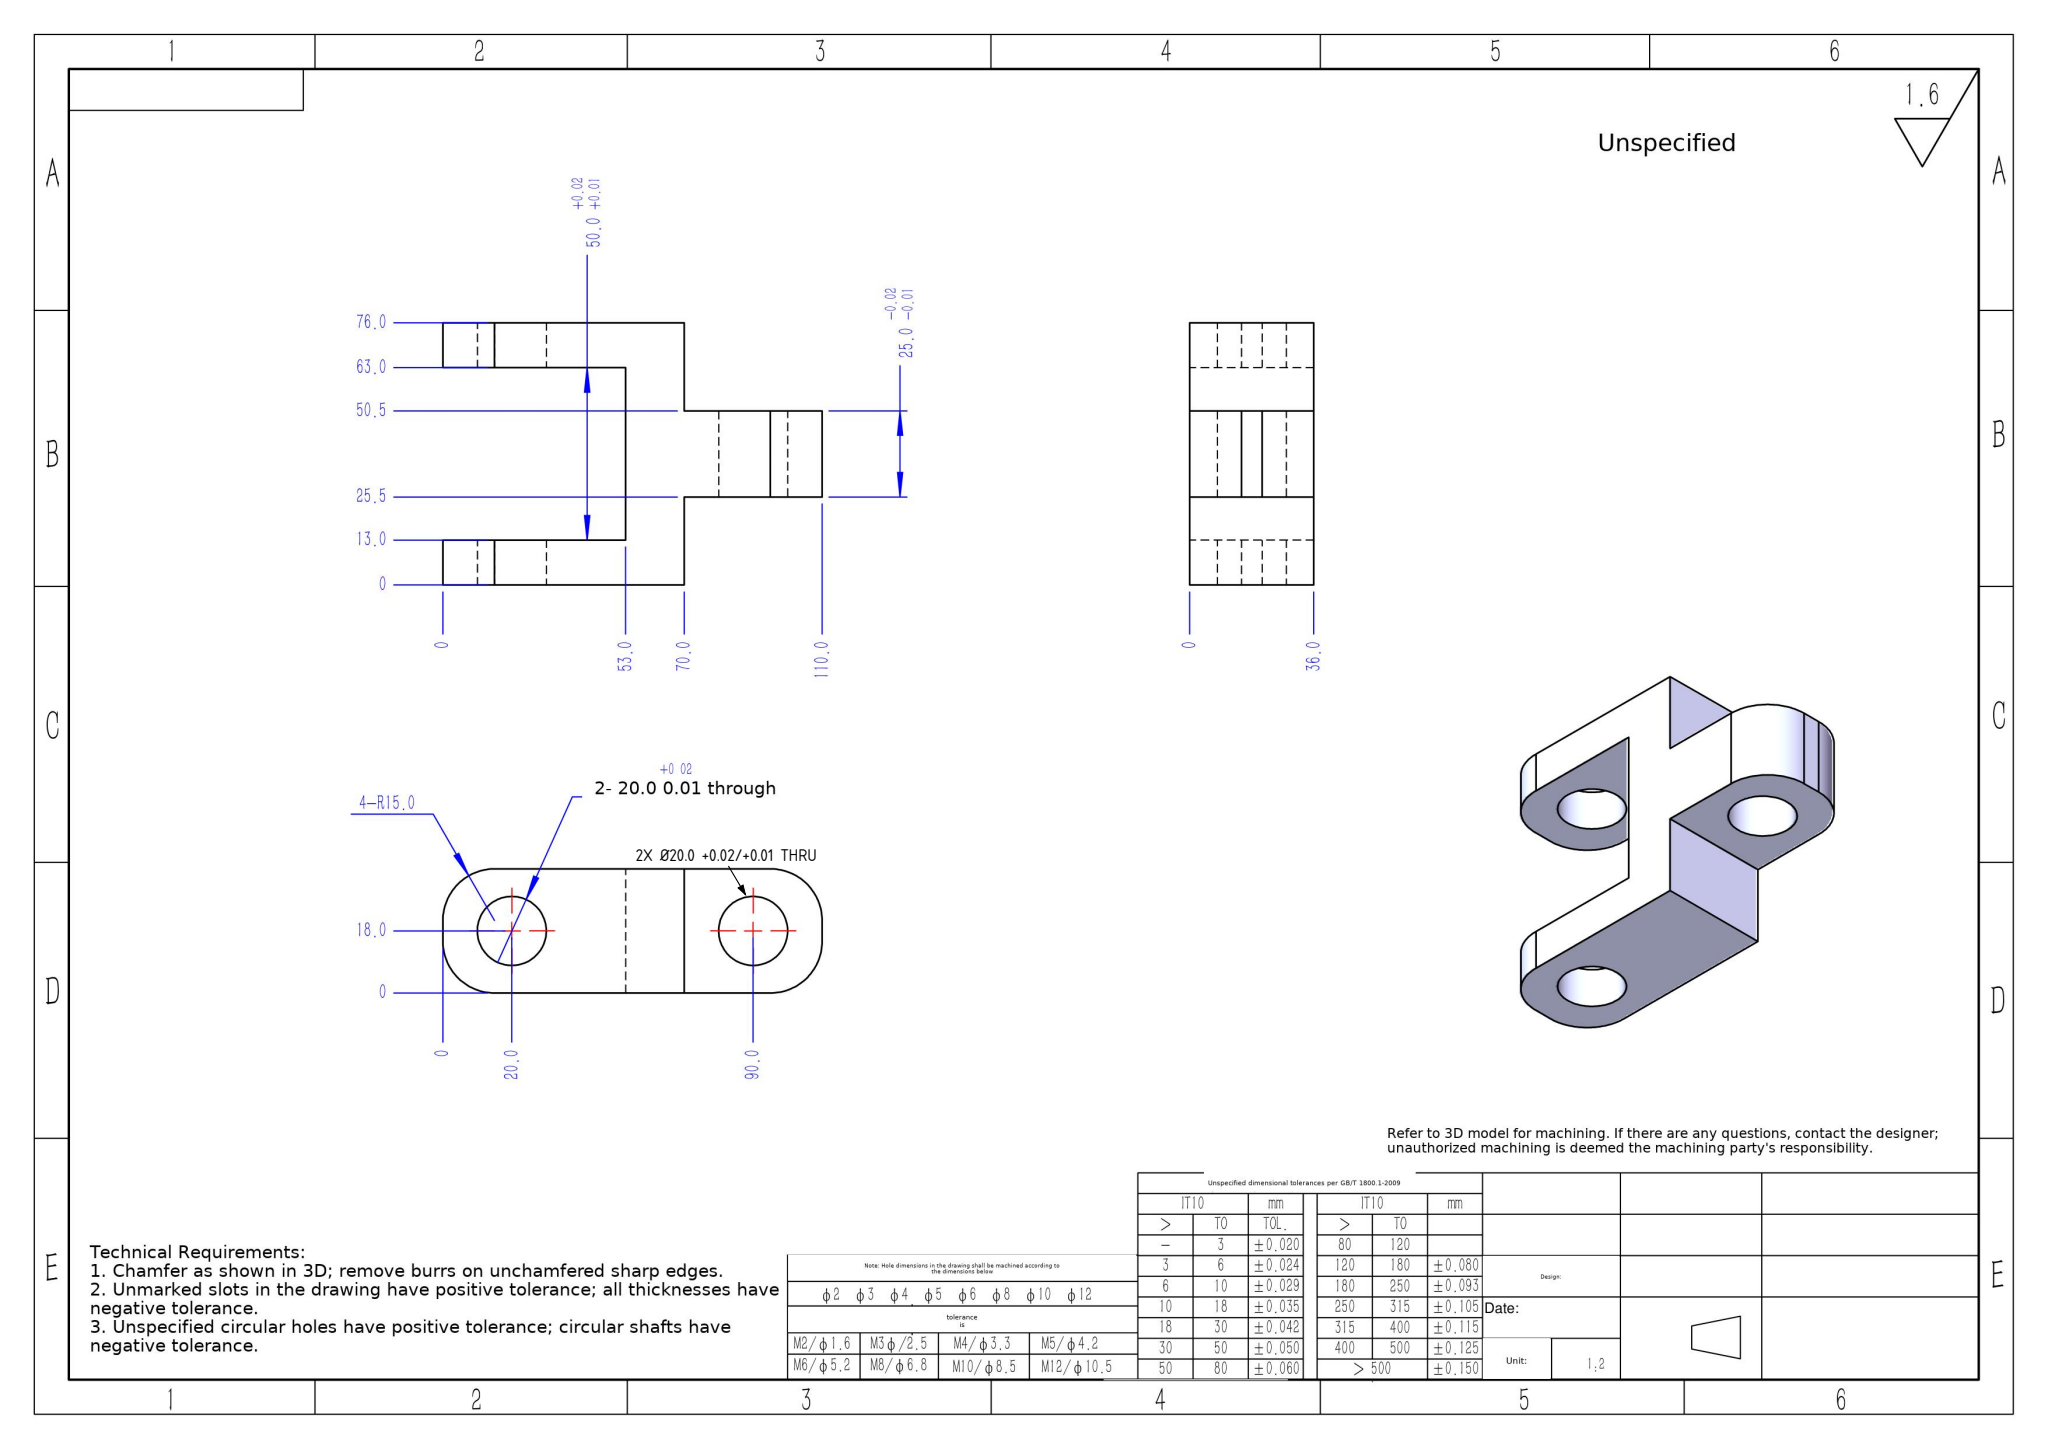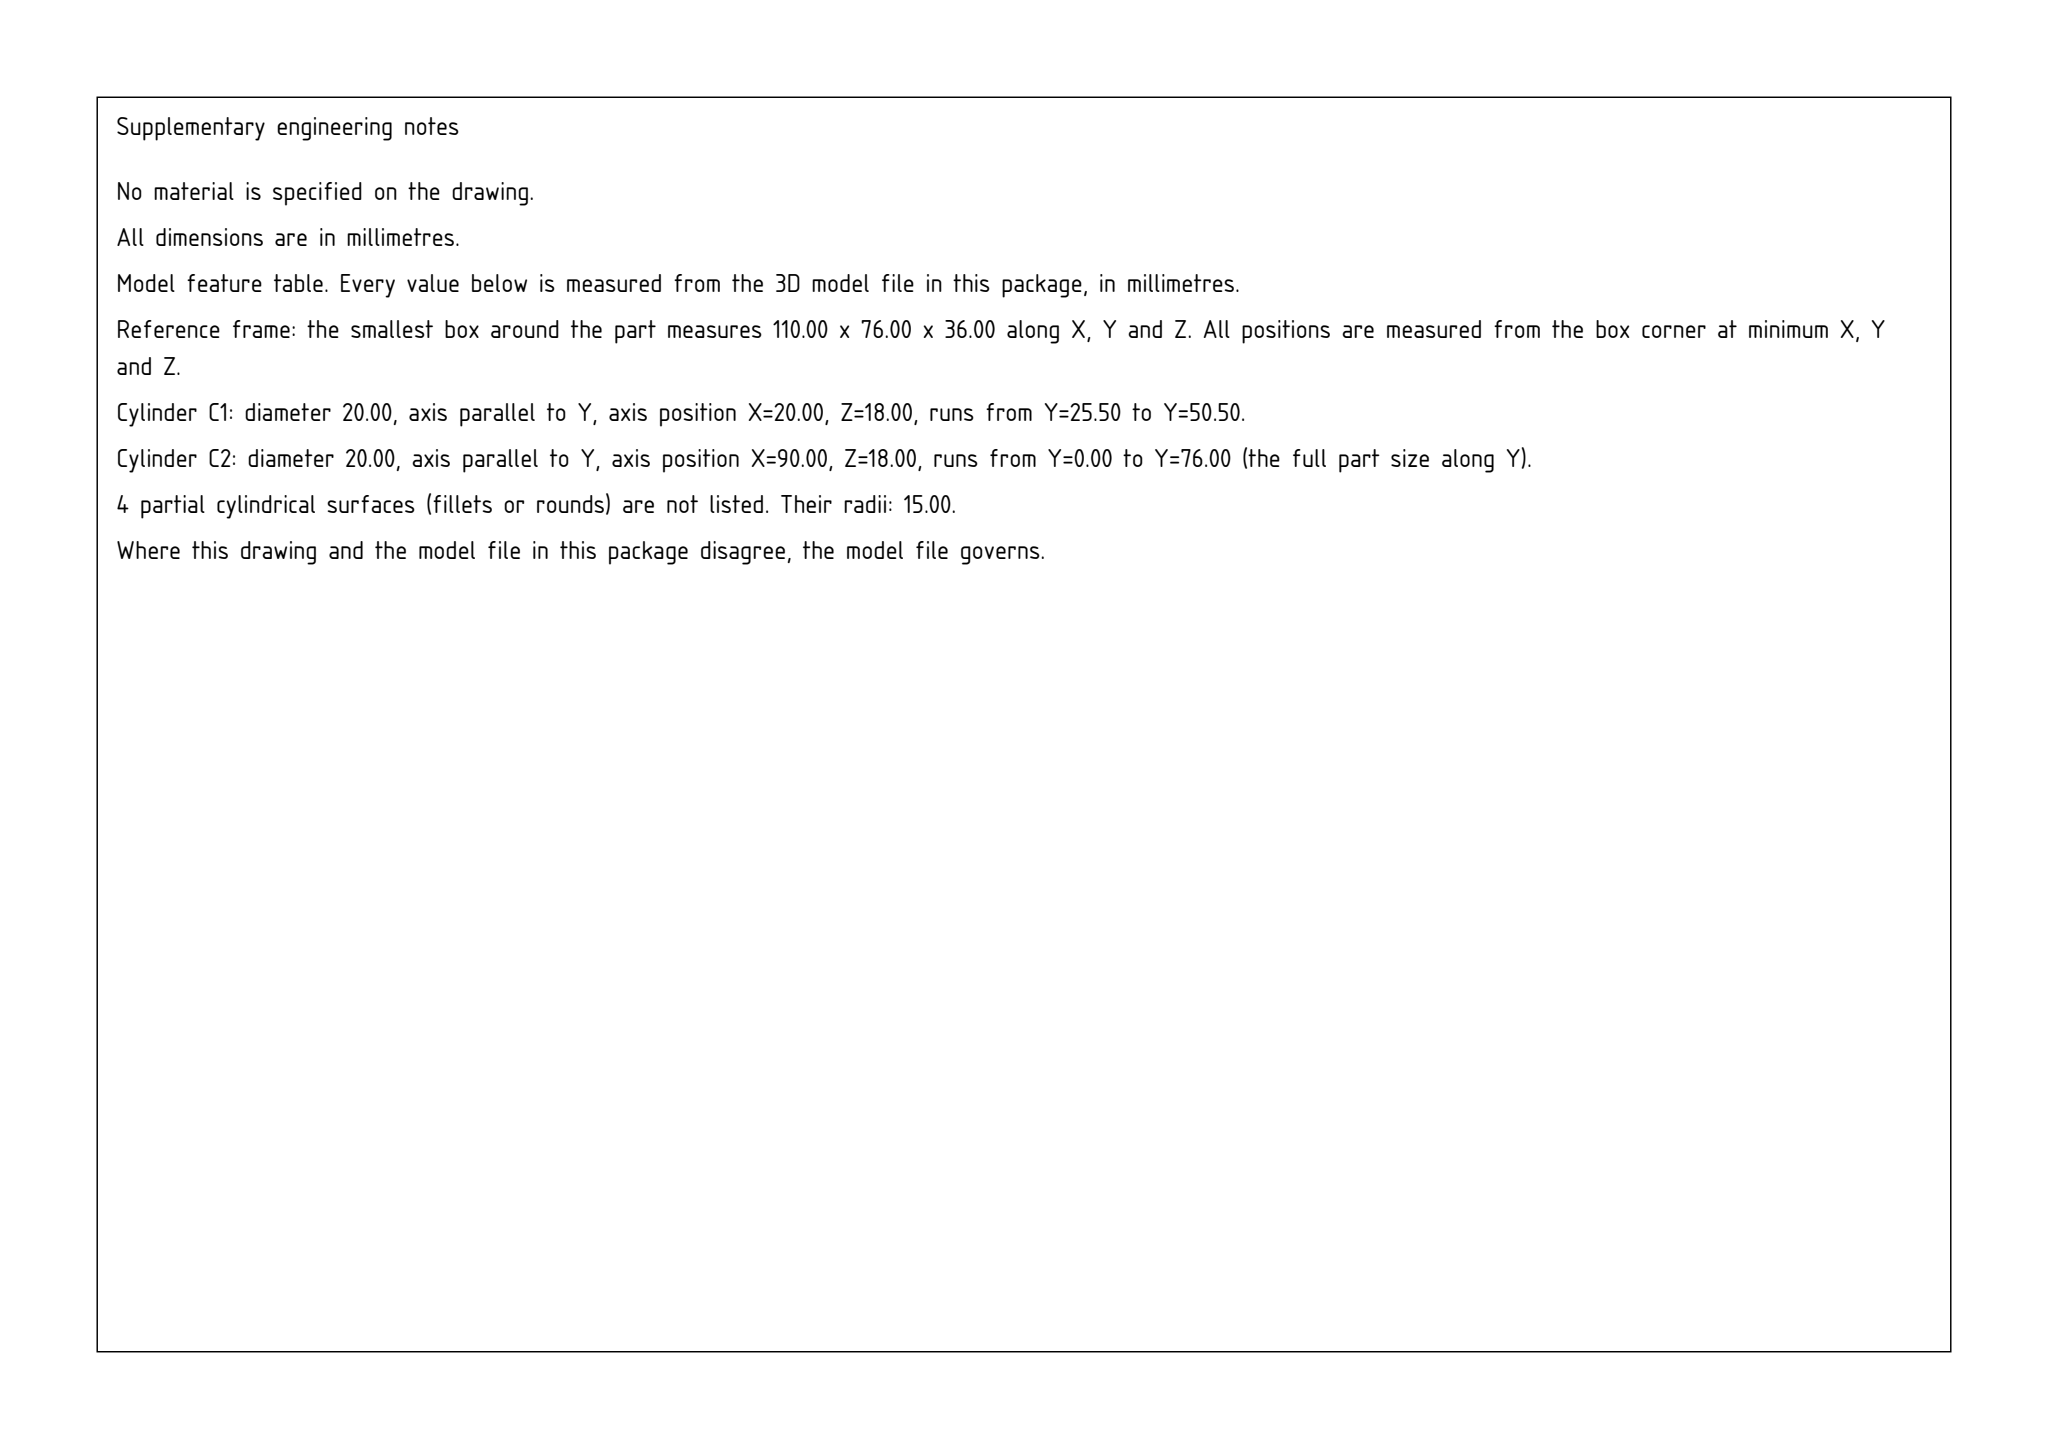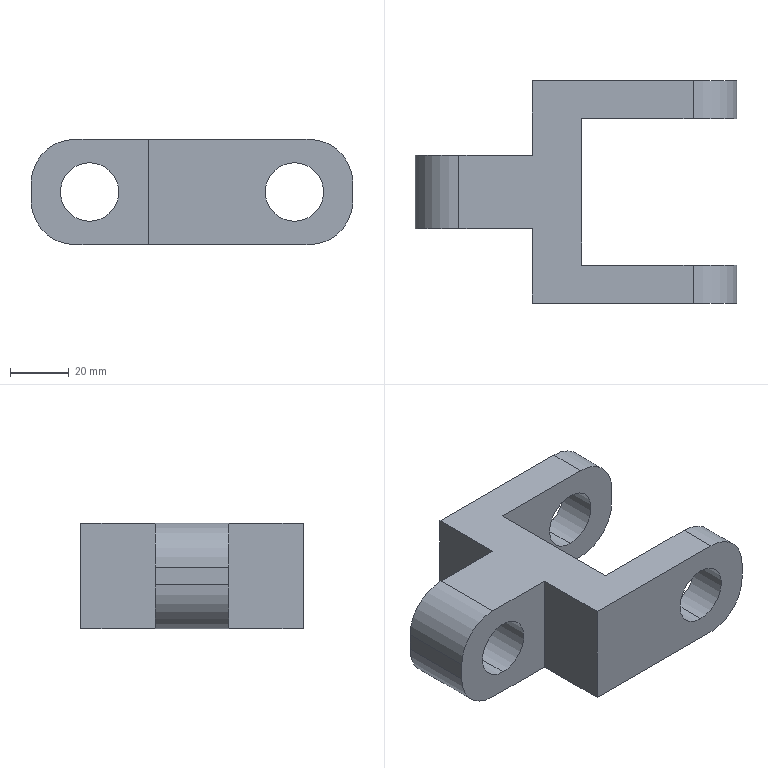Part | SolidWorks | mm | 1 solid | 26 faces | box 110 x 76 x 36 mm | volume 111173 mm3 | plane 14 | cylinder 12 | commonest cylinder face diameters 20 x6 30 x6
Drawing notes:
2X Ø20.0 +0.02/+0.01 THRU | from the solid: hole/bore dia 20.0 axis y at (x20,z18) y25.5-50.5 and (x90,z18) y0-13 & y63-76, 360 deg
build123d program:
from build123d import *

# Parameters (mm, degrees)
SKETCH1_W           = 110
SKETCH1_H           = 76
BOSS_EXTRUDE1_DEPTH = 18
SKETCH2_R           = 10
CUT_EXTRUDE1_DEPTH  = 205
SKETCH3_W           = 40
SKETCH3_H           = 36
CUT_EXTRUDE2_DEPTH  = 25.5
SKETCH4_W           = 53
SKETCH4_H           = 50
CUT_EXTRUDE3_DEPTH  = 256
FILLET1_R           = 15


with BuildPart() as part:
    # Sketch1 → Boss-Extrude1 (new, symmetric)
    with BuildSketch(Plane.XY):
        Rectangle(SKETCH1_W, SKETCH1_H)
    extrude(amount=BOSS_EXTRUDE1_DEPTH, both=True)

    # Sketch2 → Cut-Extrude1 (cut)
    with BuildSketch(Plane.XZ.offset(38)):
        with Locations(Location((35, 0, 0), (0, 0, 270))):
            Circle(SKETCH2_R)
    cut_extrude1 = extrude(amount=-CUT_EXTRUDE1_DEPTH, mode=Mode.SUBTRACT)

    # Mirror1: Cut-Extrude1 across plane
    add(cut_extrude1.mirror(Plane(origin=(0, 0, 0), x_dir=(0, 0, 1), z_dir=(1, 0, 0))), mode=Mode.SUBTRACT)

    # Sketch3 → Cut-Extrude2 (cut)
    with BuildSketch(Plane.XZ.offset(38)):
        with Locations((-35, 0)):
            Rectangle(SKETCH3_W, SKETCH3_H)
    cut_extrude2 = extrude(amount=-CUT_EXTRUDE2_DEPTH, mode=Mode.SUBTRACT)

    # Mirror2: Cut-Extrude2 across plane
    add(cut_extrude2.mirror(Plane.ZX), mode=Mode.SUBTRACT)

    # Sketch4 → Cut-Extrude3 (cut)
    with BuildSketch(Plane(origin=(0, 0, -18), x_dir=(-1, 0, 0), z_dir=(0, 0, -1))):
        with Locations((-28.5, 0)):
            Rectangle(SKETCH4_W, SKETCH4_H)
    extrude(amount=-CUT_EXTRUDE3_DEPTH, mode=Mode.SUBTRACT)

    # Fillet1
    fillet1_edges = [part.edges().sort_by_distance(p)[0] for p in [
        (55, -31.5, 18),
        (-55, 0, -18),
        (-55, 0, 18),
        (55, -31.5, -18),
        (55, 31.5, -18),
        (55, 31.5, 18),
    ]]
    fillet(fillet1_edges, radius=FILLET1_R)


solid = part.part
STEP:
#1=CARTESIAN_POINT('',(35.,-25.,-10.));
#2=VERTEX_POINT('',#1);
#3=CARTESIAN_POINT('',(35.,-25.,10.));
#4=VERTEX_POINT('',#3);
#5=CARTESIAN_POINT('',(35.,-25.,0.));
#6=DIRECTION('',(0.,1.,0.));
#7=DIRECTION('',(0.,0.,-1.));
#8=AXIS2_PLACEMENT_3D('',#5,#6,#7);
#9=CIRCLE('',#8,10.);
#10=EDGE_CURVE('',#2,#4,#9,.T.);
#11=ORIENTED_EDGE('',*,*,#10,.T.);
#12=CARTESIAN_POINT('',(35.,-38.,10.));
#13=VERTEX_POINT('',#12);
#14=CARTESIAN_POINT('',(35.,167.,10.));
#15=DIRECTION('',(0.,-1.,0.));
#16=VECTOR('',#15,1000.);
#17=LINE('',#14,#16);
#18=EDGE_CURVE('',#4,#13,#17,.T.);
#19=ORIENTED_EDGE('',*,*,#18,.T.);
#20=CARTESIAN_POINT('',(35.,-38.,-10.));
#21=VERTEX_POINT('',#20);
#22=CARTESIAN_POINT('',(35.,-38.,0.));
#23=DIRECTION('',(0.,-1.,0.));
#24=DIRECTION('',(0.,0.,-1.));
#25=AXIS2_PLACEMENT_3D('',#22,#23,#24);
#26=CIRCLE('',#25,10.);
#27=EDGE_CURVE('',#13,#21,#26,.T.);
#28=ORIENTED_EDGE('',*,*,#27,.T.);
#29=CARTESIAN_POINT('',(35.,167.,-10.));
#30=DIRECTION('',(0.,-1.,0.));
#31=VECTOR('',#30,1000.);
#32=LINE('',#29,#31);
#33=EDGE_CURVE('',#2,#21,#32,.T.);
#34=ORIENTED_EDGE('',*,*,#33,.F.);
#35=EDGE_LOOP('',(#11,#19,#28,#34));
#36=FACE_OUTER_BOUND('',#35,.T.);
#37=CARTESIAN_POINT('',(35.,167.,0.));
#38=DIRECTION('',(0.,-1.,0.));
#39=DIRECTION('',(0.,0.,-1.));
#40=AXIS2_PLACEMENT_3D('',#37,#38,#39);
#41=CYLINDRICAL_SURFACE('',#40,10.);
#42=ADVANCED_FACE('',(#36),#41,.F.);
#43=CARTESIAN_POINT('',(-35.,12.5,-10.));
#44=VERTEX_POINT('',#43);
#45=CARTESIAN_POINT('',(-35.,12.5,10.));
#46=VERTEX_POINT('',#45);
#47=CARTESIAN_POINT('',(-35.,12.5,0.));
#48=DIRECTION('',(0.,1.,0.));
#49=DIRECTION('',(0.,0.,1.));
#50=AXIS2_PLACEMENT_3D('',#47,#48,#49);
#51=CIRCLE('',#50,10.);
#52=EDGE_CURVE('',#44,#46,#51,.T.);
#53=ORIENTED_EDGE('',*,*,#52,.T.);
#54=CARTESIAN_POINT('',(-35.,-12.5,10.));
#55=VERTEX_POINT('',#54);
#56=CARTESIAN_POINT('',(-35.,167.,10.));
#57=DIRECTION('',(0.,-1.,0.));
#58=VECTOR('',#57,1000.);
#59=LINE('',#56,#58);
#60=EDGE_CURVE('',#46,#55,#59,.T.);
#61=ORIENTED_EDGE('',*,*,#60,.T.);
#62=CARTESIAN_POINT('',(-35.,-12.5,-10.));
#63=VERTEX_POINT('',#62);
#64=CARTESIAN_POINT('',(-35.,-12.5,0.));
#65=DIRECTION('',(0.,-1.,0.));
#66=DIRECTION('',(0.,0.,-1.));
#67=AXIS2_PLACEMENT_3D('',#64,#65,#66);
#68=CIRCLE('',#67,10.);
#69=EDGE_CURVE('',#55,#63,#68,.T.);
#70=ORIENTED_EDGE('',*,*,#69,.T.);
#71=CARTESIAN_POINT('',(-35.,167.,-10.));
#72=DIRECTION('',(0.,-1.,0.));
#73=VECTOR('',#72,1000.);
#74=LINE('',#71,#73);
#75=EDGE_CURVE('',#44,#63,#74,.T.);
#76=ORIENTED_EDGE('',*,*,#75,.F.);
#77=EDGE_LOOP('',(#53,#61,#70,#76));
#78=FACE_OUTER_BOUND('',#77,.T.);
#79=CARTESIAN_POINT('',(-35.,167.,0.));
#80=DIRECTION('',(0.,-1.,0.));
#81=DIRECTION('',(0.,0.,-1.));
#82=AXIS2_PLACEMENT_3D('',#79,#80,#81);
#83=CYLINDRICAL_SURFACE('',#82,10.);
#84=ADVANCED_FACE('',(#78),#83,.F.);
#85=CARTESIAN_POINT('',(35.,38.,10.));
#86=VERTEX_POINT('',#85);
#87=CARTESIAN_POINT('',(35.,38.,-10.));
#88=VERTEX_POINT('',#87);
#89=CARTESIAN_POINT('',(35.,38.,0.));
#90=DIRECTION('',(0.,-1.,0.));
#91=DIRECTION('',(0.,0.,-1.));
#92=AXIS2_PLACEMENT_3D('',#89,#90,#91);
#93=CIRCLE('',#92,10.);
#94=EDGE_CURVE('',#86,#88,#93,.T.);
#95=ORIENTED_EDGE('',*,*,#94,.F.);
#96=CARTESIAN_POINT('',(35.,25.,10.));
#97=VERTEX_POINT('',#96);
#98=CARTESIAN_POINT('',(35.,167.,10.));
#99=DIRECTION('',(0.,-1.,0.));
#100=VECTOR('',#99,1000.);
#101=LINE('',#98,#100);
#102=EDGE_CURVE('',#86,#97,#101,.T.);
#103=ORIENTED_EDGE('',*,*,#102,.T.);
#104=CARTESIAN_POINT('',(35.,25.,-10.));
#105=VERTEX_POINT('',#104);
#106=CARTESIAN_POINT('',(35.,25.,0.));
#107=DIRECTION('',(-0.,-1.,0.));
#108=DIRECTION('',(-1.,0.,0.));
#109=AXIS2_PLACEMENT_3D('',#106,#107,#108);
#110=CIRCLE('',#109,10.);
#111=EDGE_CURVE('',#97,#105,#110,.T.);
#112=ORIENTED_EDGE('',*,*,#111,.T.);
#113=CARTESIAN_POINT('',(35.,167.,-10.));
#114=DIRECTION('',(0.,-1.,0.));
#115=VECTOR('',#114,1000.);
#116=LINE('',#113,#115);
#117=EDGE_CURVE('',#88,#105,#116,.T.);
#118=ORIENTED_EDGE('',*,*,#117,.F.);
#119=EDGE_LOOP('',(#95,#103,#112,#118));
#120=FACE_OUTER_BOUND('',#119,.T.);
#121=CARTESIAN_POINT('',(35.,167.,0.));
#122=DIRECTION('',(0.,-1.,0.));
#123=DIRECTION('',(0.,0.,-1.));
#124=AXIS2_PLACEMENT_3D('',#121,#122,#123);
#125=CYLINDRICAL_SURFACE('',#124,10.);
#126=ADVANCED_FACE('',(#120),#125,.F.);
#127=CARTESIAN_POINT('',(55.,25.,3.));
#128=VERTEX_POINT('',#127);
#129=CARTESIAN_POINT('',(55.,25.,-3.));
#130=VERTEX_POINT('',#129);
#131=CARTESIAN_POINT('',(55.,25.,238.));
#132=DIRECTION('',(0.,0.,-1.));
#133=VECTOR('',#132,1000.);
#134=LINE('',#131,#133);
#135=EDGE_CURVE('',#128,#130,#134,.T.);
#136=ORIENTED_EDGE('',*,*,#135,.T.);
#137=CARTESIAN_POINT('',(55.,38.,-3.));
#138=VERTEX_POINT('',#137);
#139=CARTESIAN_POINT('',(55.,38.,-3.));
#140=DIRECTION('',(0.,1.,0.));
#141=VECTOR('',#140,1000.);
#142=LINE('',#139,#141);
#143=EDGE_CURVE('',#130,#138,#142,.T.);
#144=ORIENTED_EDGE('',*,*,#143,.T.);
#145=CARTESIAN_POINT('',(55.,38.,3.));
#146=VERTEX_POINT('',#145);
#147=CARTESIAN_POINT('',(55.,38.,18.));
#148=DIRECTION('',(0.,0.,-1.));
#149=VECTOR('',#148,1000.);
#150=LINE('',#147,#149);
#151=EDGE_CURVE('',#146,#138,#150,.T.);
#152=ORIENTED_EDGE('',*,*,#151,.F.);
#153=CARTESIAN_POINT('',(55.,-38.,3.));
#154=DIRECTION('',(0.,-1.,0.));
#155=VECTOR('',#154,1000.);
#156=LINE('',#153,#155);
#157=EDGE_CURVE('',#146,#128,#156,.T.);
#158=ORIENTED_EDGE('',*,*,#157,.T.);
#159=EDGE_LOOP('',(#136,#144,#152,#158));
#160=FACE_OUTER_BOUND('',#159,.T.);
#161=CARTESIAN_POINT('',(55.,-38.,18.));
#162=DIRECTION('',(-1.,0.,0.));
#163=DIRECTION('',(0.,0.,1.));
#164=AXIS2_PLACEMENT_3D('',#161,#162,#163);
#165=PLANE('',#164);
#166=ADVANCED_FACE('',(#160),#165,.F.);
#167=ORIENTED_EDGE('',*,*,#102,.F.);
#168=CARTESIAN_POINT('',(35.,38.,0.));
#169=DIRECTION('',(0.,-1.,0.));
#170=DIRECTION('',(0.,0.,-1.));
#171=AXIS2_PLACEMENT_3D('',#168,#169,#170);
#172=CIRCLE('',#171,10.);
#173=EDGE_CURVE('',#88,#86,#172,.T.);
#174=ORIENTED_EDGE('',*,*,#173,.F.);
#175=ORIENTED_EDGE('',*,*,#117,.T.);
#176=CARTESIAN_POINT('',(35.,25.,0.));
#177=DIRECTION('',(-0.,-1.,0.));
#178=DIRECTION('',(-1.,0.,0.));
#179=AXIS2_PLACEMENT_3D('',#176,#177,#178);
#180=CIRCLE('',#179,10.);
#181=EDGE_CURVE('',#105,#97,#180,.T.);
#182=ORIENTED_EDGE('',*,*,#181,.T.);
#183=EDGE_LOOP('',(#167,#174,#175,#182));
#184=FACE_OUTER_BOUND('',#183,.T.);
#185=CARTESIAN_POINT('',(35.,167.,0.));
#186=DIRECTION('',(0.,-1.,0.));
#187=DIRECTION('',(0.,0.,-1.));
#188=AXIS2_PLACEMENT_3D('',#185,#186,#187);
#189=CYLINDRICAL_SURFACE('',#188,10.);
#190=ADVANCED_FACE('',(#184),#189,.F.);
#191=CARTESIAN_POINT('',(-55.,12.5,3.));
#192=VERTEX_POINT('',#191);
#193=CARTESIAN_POINT('',(-55.,12.5,-3.));
#194=VERTEX_POINT('',#193);
#195=CARTESIAN_POINT('',(-55.,12.5,18.));
#196=DIRECTION('',(0.,0.,-1.));
#197=VECTOR('',#196,1000.);
#198=LINE('',#195,#197);
#199=EDGE_CURVE('',#192,#194,#198,.T.);
#200=ORIENTED_EDGE('',*,*,#199,.T.);
#201=CARTESIAN_POINT('',(-55.,-12.5,-3.));
#202=VERTEX_POINT('',#201);
#203=CARTESIAN_POINT('',(-55.,-12.5,-3.));
#204=DIRECTION('',(0.,-1.,0.));
#205=VECTOR('',#204,1000.);
#206=LINE('',#203,#205);
#207=EDGE_CURVE('',#194,#202,#206,.T.);
#208=ORIENTED_EDGE('',*,*,#207,.T.);
#209=CARTESIAN_POINT('',(-55.,-12.5,3.));
#210=VERTEX_POINT('',#209);
#211=CARTESIAN_POINT('',(-55.,-12.5,18.));
#212=DIRECTION('',(0.,0.,-1.));
#213=VECTOR('',#212,1000.);
#214=LINE('',#211,#213);
#215=EDGE_CURVE('',#210,#202,#214,.T.);
#216=ORIENTED_EDGE('',*,*,#215,.F.);
#217=CARTESIAN_POINT('',(-55.,-38.,3.));
#218=DIRECTION('',(0.,1.,0.));
#219=VECTOR('',#218,1000.);
#220=LINE('',#217,#219);
#221=EDGE_CURVE('',#210,#192,#220,.T.);
#222=ORIENTED_EDGE('',*,*,#221,.T.);
#223=EDGE_LOOP('',(#200,#208,#216,#222));
#224=FACE_OUTER_BOUND('',#223,.T.);
#225=CARTESIAN_POINT('',(-55.,-38.,18.));
#226=DIRECTION('',(1.,0.,0.));
#227=DIRECTION('',(0.,0.,-1.));
#228=AXIS2_PLACEMENT_3D('',#225,#226,#227);
#229=PLANE('',#228);
#230=ADVANCED_FACE('',(#224),#229,.F.);
#231=ORIENTED_EDGE('',*,*,#60,.F.);
#232=CARTESIAN_POINT('',(-35.,12.5,0.));
#233=DIRECTION('',(0.,1.,0.));
#234=DIRECTION('',(0.,0.,1.));
#235=AXIS2_PLACEMENT_3D('',#232,#233,#234);
#236=CIRCLE('',#235,10.);
#237=EDGE_CURVE('',#46,#44,#236,.T.);
#238=ORIENTED_EDGE('',*,*,#237,.T.);
#239=ORIENTED_EDGE('',*,*,#75,.T.);
#240=CARTESIAN_POINT('',(-35.,-12.5,0.));
#241=DIRECTION('',(0.,-1.,0.));
#242=DIRECTION('',(0.,0.,-1.));
#243=AXIS2_PLACEMENT_3D('',#240,#241,#242);
#244=CIRCLE('',#243,10.);
#245=EDGE_CURVE('',#63,#55,#244,.T.);
#246=ORIENTED_EDGE('',*,*,#245,.T.);
#247=EDGE_LOOP('',(#231,#238,#239,#246));
#248=FACE_OUTER_BOUND('',#247,.T.);
#249=CARTESIAN_POINT('',(-35.,167.,0.));
#250=DIRECTION('',(0.,-1.,0.));
#251=DIRECTION('',(0.,0.,-1.));
#252=AXIS2_PLACEMENT_3D('',#249,#250,#251);
#253=CYLINDRICAL_SURFACE('',#252,10.);
#254=ADVANCED_FACE('',(#248),#253,.F.);
#255=ORIENTED_EDGE('',*,*,#173,.T.);
#256=ORIENTED_EDGE('',*,*,#94,.T.);
#257=EDGE_LOOP('',(#255,#256));
#258=FACE_BOUND('',#257,.T.);
#259=ORIENTED_EDGE('',*,*,#151,.T.);
#260=CARTESIAN_POINT('',(40.,38.,-18.));
#261=VERTEX_POINT('',#260);
#262=CARTESIAN_POINT('',(40.,38.,-3.));
#263=DIRECTION('',(0.,1.,0.));
#264=DIRECTION('',(0.,0.,-1.));
#265=AXIS2_PLACEMENT_3D('',#262,#263,#264);
#266=CIRCLE('',#265,15.);
#267=EDGE_CURVE('',#138,#261,#266,.T.);
#268=ORIENTED_EDGE('',*,*,#267,.T.);
#269=CARTESIAN_POINT('',(-15.,38.,-18.));
#270=VERTEX_POINT('',#269);
#271=CARTESIAN_POINT('',(-55.,38.,-18.));
#272=DIRECTION('',(-1.,0.,0.));
#273=VECTOR('',#272,1000.);
#274=LINE('',#271,#273);
#275=EDGE_CURVE('',#261,#270,#274,.T.);
#276=ORIENTED_EDGE('',*,*,#275,.T.);
#277=CARTESIAN_POINT('',(-15.,38.,18.));
#278=VERTEX_POINT('',#277);
#279=CARTESIAN_POINT('',(-15.,38.,18.));
#280=DIRECTION('',(-0.,0.,1.));
#281=VECTOR('',#280,1000.);
#282=LINE('',#279,#281);
#283=EDGE_CURVE('',#270,#278,#282,.T.);
#284=ORIENTED_EDGE('',*,*,#283,.T.);
#285=CARTESIAN_POINT('',(40.,38.,18.));
#286=VERTEX_POINT('',#285);
#287=CARTESIAN_POINT('',(-55.,38.,18.));
#288=DIRECTION('',(-1.,0.,0.));
#289=VECTOR('',#288,1000.);
#290=LINE('',#287,#289);
#291=EDGE_CURVE('',#286,#278,#290,.T.);
#292=ORIENTED_EDGE('',*,*,#291,.F.);
#293=CARTESIAN_POINT('',(40.,38.,3.));
#294=DIRECTION('',(0.,1.,0.));
#295=DIRECTION('',(0.,0.,-1.));
#296=AXIS2_PLACEMENT_3D('',#293,#294,#295);
#297=CIRCLE('',#296,15.);
#298=EDGE_CURVE('',#286,#146,#297,.T.);
#299=ORIENTED_EDGE('',*,*,#298,.T.);
#300=EDGE_LOOP('',(#259,#268,#276,#284,#292,#299));
#301=FACE_OUTER_BOUND('',#300,.T.);
#302=CARTESIAN_POINT('',(-55.,38.,18.));
#303=DIRECTION('',(0.,-1.,0.));
#304=DIRECTION('',(0.,0.,-1.));
#305=AXIS2_PLACEMENT_3D('',#302,#303,#304);
#306=PLANE('',#305);
#307=ADVANCED_FACE('',(#258,#301),#306,.F.);
#308=CARTESIAN_POINT('',(-15.,12.5,18.));
#309=VERTEX_POINT('',#308);
#310=CARTESIAN_POINT('',(-40.,12.5,18.));
#311=VERTEX_POINT('',#310);
#312=CARTESIAN_POINT('',(-55.,12.5,18.));
#313=DIRECTION('',(-1.,0.,0.));
#314=VECTOR('',#313,1000.);
#315=LINE('',#312,#314);
#316=EDGE_CURVE('',#309,#311,#315,.T.);
#317=ORIENTED_EDGE('',*,*,#316,.T.);
#318=CARTESIAN_POINT('',(-40.,-12.5,18.));
#319=VERTEX_POINT('',#318);
#320=CARTESIAN_POINT('',(-40.,0.,18.));
#321=DIRECTION('',(0.,-1.,0.));
#322=VECTOR('',#321,1000.);
#323=LINE('',#320,#322);
#324=EDGE_CURVE('',#311,#319,#323,.T.);
#325=ORIENTED_EDGE('',*,*,#324,.T.);
#326=CARTESIAN_POINT('',(-15.,-12.5,18.));
#327=VERTEX_POINT('',#326);
#328=CARTESIAN_POINT('',(-55.,-12.5,18.));
#329=DIRECTION('',(-1.,0.,0.));
#330=VECTOR('',#329,1000.);
#331=LINE('',#328,#330);
#332=EDGE_CURVE('',#327,#319,#331,.T.);
#333=ORIENTED_EDGE('',*,*,#332,.F.);
#334=CARTESIAN_POINT('',(-15.,-38.,18.));
#335=VERTEX_POINT('',#334);
#336=CARTESIAN_POINT('',(-15.,-12.5,18.));
#337=DIRECTION('',(0.,-1.,0.));
#338=VECTOR('',#337,1000.);
#339=LINE('',#336,#338);
#340=EDGE_CURVE('',#327,#335,#339,.T.);
#341=ORIENTED_EDGE('',*,*,#340,.T.);
#342=CARTESIAN_POINT('',(40.,-38.,18.));
#343=VERTEX_POINT('',#342);
#344=CARTESIAN_POINT('',(-55.,-38.,18.));
#345=DIRECTION('',(1.,0.,0.));
#346=VECTOR('',#345,1000.);
#347=LINE('',#344,#346);
#348=EDGE_CURVE('',#335,#343,#347,.T.);
#349=ORIENTED_EDGE('',*,*,#348,.T.);
#350=CARTESIAN_POINT('',(40.,-25.,18.));
#351=VERTEX_POINT('',#350);
#352=CARTESIAN_POINT('',(40.,0.,18.));
#353=DIRECTION('',(0.,1.,0.));
#354=VECTOR('',#353,1000.);
#355=LINE('',#352,#354);
#356=EDGE_CURVE('',#343,#351,#355,.T.);
#357=ORIENTED_EDGE('',*,*,#356,.T.);
#358=CARTESIAN_POINT('',(2.,-25.,18.));
#359=VERTEX_POINT('',#358);
#360=CARTESIAN_POINT('',(0.,-25.,18.));
#361=DIRECTION('',(-1.,0.,0.));
#362=VECTOR('',#361,1000.);
#363=LINE('',#360,#362);
#364=EDGE_CURVE('',#351,#359,#363,.T.);
#365=ORIENTED_EDGE('',*,*,#364,.T.);
#366=CARTESIAN_POINT('',(2.,25.,18.));
#367=VERTEX_POINT('',#366);
#368=CARTESIAN_POINT('',(2.,-0.,18.));
#369=DIRECTION('',(0.,1.,0.));
#370=VECTOR('',#369,1000.);
#371=LINE('',#368,#370);
#372=EDGE_CURVE('',#359,#367,#371,.T.);
#373=ORIENTED_EDGE('',*,*,#372,.T.);
#374=CARTESIAN_POINT('',(40.,25.,18.));
#375=VERTEX_POINT('',#374);
#376=CARTESIAN_POINT('',(0.,25.,18.));
#377=DIRECTION('',(1.,-0.,0.));
#378=VECTOR('',#377,1000.);
#379=LINE('',#376,#378);
#380=EDGE_CURVE('',#367,#375,#379,.T.);
#381=ORIENTED_EDGE('',*,*,#380,.T.);
#382=CARTESIAN_POINT('',(40.,0.,18.));
#383=DIRECTION('',(0.,1.,0.));
#384=VECTOR('',#383,1000.);
#385=LINE('',#382,#384);
#386=EDGE_CURVE('',#375,#286,#385,.T.);
#387=ORIENTED_EDGE('',*,*,#386,.T.);
#388=ORIENTED_EDGE('',*,*,#291,.T.);
#389=CARTESIAN_POINT('',(-15.,12.5,18.));
#390=DIRECTION('',(0.,1.,0.));
#391=VECTOR('',#390,1000.);
#392=LINE('',#389,#391);
#393=EDGE_CURVE('',#309,#278,#392,.T.);
#394=ORIENTED_EDGE('',*,*,#393,.F.);
#395=EDGE_LOOP('',(#317,#325,#333,#341,#349,#357,#365,#373,#381,#387,#388,#394));
#396=FACE_OUTER_BOUND('',#395,.T.);
#397=CARTESIAN_POINT('',(0.,0.,18.));
#398=DIRECTION('',(0.,0.,-1.));
#399=DIRECTION('',(-1.,0.,0.));
#400=AXIS2_PLACEMENT_3D('',#397,#398,#399);
#401=PLANE('',#400);
#402=ADVANCED_FACE('',(#396),#401,.F.);
#403=CARTESIAN_POINT('',(-40.,-12.5,-18.));
#404=VERTEX_POINT('',#403);
#405=CARTESIAN_POINT('',(-15.,-12.5,-18.));
#406=VERTEX_POINT('',#405);
#407=CARTESIAN_POINT('',(-55.,-12.5,-18.));
#408=DIRECTION('',(1.,0.,0.));
#409=VECTOR('',#408,1000.);
#410=LINE('',#407,#409);
#411=EDGE_CURVE('',#404,#406,#410,.T.);
#412=ORIENTED_EDGE('',*,*,#411,.F.);
#413=CARTESIAN_POINT('',(-40.,12.5,-18.));
#414=VERTEX_POINT('',#413);
#415=CARTESIAN_POINT('',(-40.,12.5,-18.));
#416=DIRECTION('',(0.,1.,0.));
#417=VECTOR('',#416,1000.);
#418=LINE('',#415,#417);
#419=EDGE_CURVE('',#404,#414,#418,.T.);
#420=ORIENTED_EDGE('',*,*,#419,.T.);
#421=CARTESIAN_POINT('',(-15.,12.5,-18.));
#422=VERTEX_POINT('',#421);
#423=CARTESIAN_POINT('',(-55.,12.5,-18.));
#424=DIRECTION('',(1.,0.,0.));
#425=VECTOR('',#424,1000.);
#426=LINE('',#423,#425);
#427=EDGE_CURVE('',#414,#422,#426,.T.);
#428=ORIENTED_EDGE('',*,*,#427,.T.);
#429=CARTESIAN_POINT('',(-15.,12.5,-18.));
#430=DIRECTION('',(0.,1.,0.));
#431=VECTOR('',#430,1000.);
#432=LINE('',#429,#431);
#433=EDGE_CURVE('',#422,#270,#432,.T.);
#434=ORIENTED_EDGE('',*,*,#433,.T.);
#435=ORIENTED_EDGE('',*,*,#275,.F.);
#436=CARTESIAN_POINT('',(40.,25.,-18.));
#437=VERTEX_POINT('',#436);
#438=CARTESIAN_POINT('',(40.,25.,-18.));
#439=DIRECTION('',(0.,-1.,0.));
#440=VECTOR('',#439,1000.);
#441=LINE('',#438,#440);
#442=EDGE_CURVE('',#261,#437,#441,.T.);
#443=ORIENTED_EDGE('',*,*,#442,.T.);
#444=CARTESIAN_POINT('',(2.,25.,-18.));
#445=VERTEX_POINT('',#444);
#446=CARTESIAN_POINT('',(55.,25.,-18.));
#447=DIRECTION('',(1.,-0.,0.));
#448=VECTOR('',#447,1000.);
#449=LINE('',#446,#448);
#450=EDGE_CURVE('',#445,#437,#449,.T.);
#451=ORIENTED_EDGE('',*,*,#450,.F.);
#452=CARTESIAN_POINT('',(2.,-25.,-18.));
#453=VERTEX_POINT('',#452);
#454=CARTESIAN_POINT('',(2.,-25.,-18.));
#455=DIRECTION('',(0.,1.,0.));
#456=VECTOR('',#455,1000.);
#457=LINE('',#454,#456);
#458=EDGE_CURVE('',#453,#445,#457,.T.);
#459=ORIENTED_EDGE('',*,*,#458,.F.);
#460=CARTESIAN_POINT('',(40.,-25.,-18.));
#461=VERTEX_POINT('',#460);
#462=CARTESIAN_POINT('',(55.,-25.,-18.));
#463=DIRECTION('',(-1.,0.,0.));
#464=VECTOR('',#463,1000.);
#465=LINE('',#462,#464);
#466=EDGE_CURVE('',#461,#453,#465,.T.);
#467=ORIENTED_EDGE('',*,*,#466,.F.);
#468=CARTESIAN_POINT('',(40.,-38.,-18.));
#469=VERTEX_POINT('',#468);
#470=CARTESIAN_POINT('',(40.,-38.,-18.));
#471=DIRECTION('',(0.,-1.,0.));
#472=VECTOR('',#471,1000.);
#473=LINE('',#470,#472);
#474=EDGE_CURVE('',#461,#469,#473,.T.);
#475=ORIENTED_EDGE('',*,*,#474,.T.);
#476=CARTESIAN_POINT('',(-15.,-38.,-18.));
#477=VERTEX_POINT('',#476);
#478=CARTESIAN_POINT('',(-55.,-38.,-18.));
#479=DIRECTION('',(1.,0.,0.));
#480=VECTOR('',#479,1000.);
#481=LINE('',#478,#480);
#482=EDGE_CURVE('',#477,#469,#481,.T.);
#483=ORIENTED_EDGE('',*,*,#482,.F.);
#484=CARTESIAN_POINT('',(-15.,-12.5,-18.));
#485=DIRECTION('',(0.,-1.,0.));
#486=VECTOR('',#485,1000.);
#487=LINE('',#484,#486);
#488=EDGE_CURVE('',#406,#477,#487,.T.);
#489=ORIENTED_EDGE('',*,*,#488,.F.);
#490=EDGE_LOOP('',(#412,#420,#428,#434,#435,#443,#451,#459,#467,#475,#483,#489));
#491=FACE_OUTER_BOUND('',#490,.T.);
#492=CARTESIAN_POINT('',(0.,0.,-18.));
#493=DIRECTION('',(0.,0.,-1.));
#494=DIRECTION('',(-1.,0.,0.));
#495=AXIS2_PLACEMENT_3D('',#492,#493,#494);
#496=PLANE('',#495);
#497=ADVANCED_FACE('',(#491),#496,.T.);
#498=CARTESIAN_POINT('',(55.,-38.,3.));
#499=VERTEX_POINT('',#498);
#500=CARTESIAN_POINT('',(55.,-38.,-3.));
#501=VERTEX_POINT('',#500);
#502=CARTESIAN_POINT('',(55.,-38.,18.));
#503=DIRECTION('',(0.,0.,-1.));
#504=VECTOR('',#503,1000.);
#505=LINE('',#502,#504);
#506=EDGE_CURVE('',#499,#501,#505,.T.);
#507=ORIENTED_EDGE('',*,*,#506,.T.);
#508=CARTESIAN_POINT('',(55.,-25.,-3.));
#509=VERTEX_POINT('',#508);
#510=CARTESIAN_POINT('',(55.,-25.,-3.));
#511=DIRECTION('',(0.,1.,0.));
#512=VECTOR('',#511,1000.);
#513=LINE('',#510,#512);
#514=EDGE_CURVE('',#501,#509,#513,.T.);
#515=ORIENTED_EDGE('',*,*,#514,.T.);
#516=CARTESIAN_POINT('',(55.,-25.,3.));
#517=VERTEX_POINT('',#516);
#518=CARTESIAN_POINT('',(55.,-25.,238.));
#519=DIRECTION('',(0.,0.,-1.));
#520=VECTOR('',#519,1000.);
#521=LINE('',#518,#520);
#522=EDGE_CURVE('',#517,#509,#521,.T.);
#523=ORIENTED_EDGE('',*,*,#522,.F.);
#524=CARTESIAN_POINT('',(55.,-38.,3.));
#525=DIRECTION('',(0.,-1.,0.));
#526=VECTOR('',#525,1000.);
#527=LINE('',#524,#526);
#528=EDGE_CURVE('',#517,#499,#527,.T.);
#529=ORIENTED_EDGE('',*,*,#528,.T.);
#530=EDGE_LOOP('',(#507,#515,#523,#529));
#531=FACE_OUTER_BOUND('',#530,.T.);
#532=CARTESIAN_POINT('',(55.,-38.,18.));
#533=DIRECTION('',(-1.,0.,0.));
#534=DIRECTION('',(0.,0.,1.));
#535=AXIS2_PLACEMENT_3D('',#532,#533,#534);
#536=PLANE('',#535);
#537=ADVANCED_FACE('',(#531),#536,.F.);
#538=CARTESIAN_POINT('',(35.,-38.,0.));
#539=DIRECTION('',(0.,-1.,0.));
#540=DIRECTION('',(0.,0.,-1.));
#541=AXIS2_PLACEMENT_3D('',#538,#539,#540);
#542=CIRCLE('',#541,10.);
#543=EDGE_CURVE('',#21,#13,#542,.T.);
#544=ORIENTED_EDGE('',*,*,#543,.F.);
#545=ORIENTED_EDGE('',*,*,#27,.F.);
#546=EDGE_LOOP('',(#544,#545));
#547=FACE_BOUND('',#546,.T.);
#548=ORIENTED_EDGE('',*,*,#482,.T.);
#549=CARTESIAN_POINT('',(40.,-38.,-3.));
#550=DIRECTION('',(0.,-1.,0.));
#551=DIRECTION('',(0.,0.,1.));
#552=AXIS2_PLACEMENT_3D('',#549,#550,#551);
#553=CIRCLE('',#552,15.);
#554=EDGE_CURVE('',#469,#501,#553,.T.);
#555=ORIENTED_EDGE('',*,*,#554,.T.);
#556=ORIENTED_EDGE('',*,*,#506,.F.);
#557=CARTESIAN_POINT('',(40.,-38.,3.));
#558=DIRECTION('',(0.,-1.,0.));
#559=DIRECTION('',(0.,0.,1.));
#560=AXIS2_PLACEMENT_3D('',#557,#558,#559);
#561=CIRCLE('',#560,15.);
#562=EDGE_CURVE('',#499,#343,#561,.T.);
#563=ORIENTED_EDGE('',*,*,#562,.T.);
#564=ORIENTED_EDGE('',*,*,#348,.F.);
#565=CARTESIAN_POINT('',(-15.,-38.,18.));
#566=DIRECTION('',(-0.,0.,1.));
#567=VECTOR('',#566,1000.);
#568=LINE('',#565,#567);
#569=EDGE_CURVE('',#477,#335,#568,.T.);
#570=ORIENTED_EDGE('',*,*,#569,.F.);
#571=EDGE_LOOP('',(#548,#555,#556,#563,#564,#570));
#572=FACE_OUTER_BOUND('',#571,.T.);
#573=CARTESIAN_POINT('',(-55.,-38.,18.));
#574=DIRECTION('',(0.,1.,0.));
#575=DIRECTION('',(0.,0.,1.));
#576=AXIS2_PLACEMENT_3D('',#573,#574,#575);
#577=PLANE('',#576);
#578=ADVANCED_FACE('',(#547,#572),#577,.F.);
#579=ORIENTED_EDGE('',*,*,#18,.F.);
#580=CARTESIAN_POINT('',(35.,-25.,0.));
#581=DIRECTION('',(0.,1.,0.));
#582=DIRECTION('',(0.,0.,-1.));
#583=AXIS2_PLACEMENT_3D('',#580,#581,#582);
#584=CIRCLE('',#583,10.);
#585=EDGE_CURVE('',#4,#2,#584,.T.);
#586=ORIENTED_EDGE('',*,*,#585,.T.);
#587=ORIENTED_EDGE('',*,*,#33,.T.);
#588=ORIENTED_EDGE('',*,*,#543,.T.);
#589=EDGE_LOOP('',(#579,#586,#587,#588));
#590=FACE_OUTER_BOUND('',#589,.T.);
#591=CARTESIAN_POINT('',(35.,167.,0.));
#592=DIRECTION('',(0.,-1.,0.));
#593=DIRECTION('',(0.,0.,-1.));
#594=AXIS2_PLACEMENT_3D('',#591,#592,#593);
#595=CYLINDRICAL_SURFACE('',#594,10.);
#596=ADVANCED_FACE('',(#590),#595,.F.);
#597=ORIENTED_EDGE('',*,*,#569,.T.);
#598=ORIENTED_EDGE('',*,*,#340,.F.);
#599=CARTESIAN_POINT('',(-15.,-12.5,18.));
#600=DIRECTION('',(-0.,0.,1.));
#601=VECTOR('',#600,1000.);
#602=LINE('',#599,#601);
#603=EDGE_CURVE('',#406,#327,#602,.T.);
#604=ORIENTED_EDGE('',*,*,#603,.F.);
#605=ORIENTED_EDGE('',*,*,#488,.T.);
#606=EDGE_LOOP('',(#597,#598,#604,#605));
#607=FACE_OUTER_BOUND('',#606,.T.);
#608=CARTESIAN_POINT('',(-15.,-12.5,18.));
#609=DIRECTION('',(1.,0.,0.));
#610=DIRECTION('',(0.,0.,-1.));
#611=AXIS2_PLACEMENT_3D('',#608,#609,#610);
#612=PLANE('',#611);
#613=ADVANCED_FACE('',(#607),#612,.F.);
#614=ORIENTED_EDGE('',*,*,#245,.F.);
#615=ORIENTED_EDGE('',*,*,#69,.F.);
#616=EDGE_LOOP('',(#614,#615));
#617=FACE_BOUND('',#616,.T.);
#618=ORIENTED_EDGE('',*,*,#215,.T.);
#619=CARTESIAN_POINT('',(-40.,-12.5,-3.));
#620=DIRECTION('',(0.,-1.,0.));
#621=DIRECTION('',(0.,0.,-1.));
#622=AXIS2_PLACEMENT_3D('',#619,#620,#621);
#623=CIRCLE('',#622,15.);
#624=EDGE_CURVE('',#202,#404,#623,.T.);
#625=ORIENTED_EDGE('',*,*,#624,.T.);
#626=ORIENTED_EDGE('',*,*,#411,.T.);
#627=ORIENTED_EDGE('',*,*,#603,.T.);
#628=ORIENTED_EDGE('',*,*,#332,.T.);
#629=CARTESIAN_POINT('',(-40.,-12.5,3.));
#630=DIRECTION('',(0.,-1.,0.));
#631=DIRECTION('',(0.,0.,-1.));
#632=AXIS2_PLACEMENT_3D('',#629,#630,#631);
#633=CIRCLE('',#632,15.);
#634=EDGE_CURVE('',#319,#210,#633,.T.);
#635=ORIENTED_EDGE('',*,*,#634,.T.);
#636=EDGE_LOOP('',(#618,#625,#626,#627,#628,#635));
#637=FACE_OUTER_BOUND('',#636,.T.);
#638=CARTESIAN_POINT('',(0.,-12.5,0.));
#639=DIRECTION('',(0.,-1.,0.));
#640=DIRECTION('',(0.,0.,-1.));
#641=AXIS2_PLACEMENT_3D('',#638,#639,#640);
#642=PLANE('',#641);
#643=ADVANCED_FACE('',(#617,#637),#642,.T.);
#644=ORIENTED_EDGE('',*,*,#283,.F.);
#645=ORIENTED_EDGE('',*,*,#433,.F.);
#646=CARTESIAN_POINT('',(-15.,12.5,18.));
#647=DIRECTION('',(-0.,0.,1.));
#648=VECTOR('',#647,1000.);
#649=LINE('',#646,#648);
#650=EDGE_CURVE('',#422,#309,#649,.T.);
#651=ORIENTED_EDGE('',*,*,#650,.T.);
#652=ORIENTED_EDGE('',*,*,#393,.T.);
#653=EDGE_LOOP('',(#644,#645,#651,#652));
#654=FACE_OUTER_BOUND('',#653,.T.);
#655=CARTESIAN_POINT('',(-15.,12.5,18.));
#656=DIRECTION('',(-1.,0.,-0.));
#657=DIRECTION('',(-0.,0.,1.));
#658=AXIS2_PLACEMENT_3D('',#655,#656,#657);
#659=PLANE('',#658);
#660=ADVANCED_FACE('',(#654),#659,.T.);
#661=ORIENTED_EDGE('',*,*,#52,.F.);
#662=ORIENTED_EDGE('',*,*,#237,.F.);
#663=EDGE_LOOP('',(#661,#662));
#664=FACE_BOUND('',#663,.T.);
#665=ORIENTED_EDGE('',*,*,#427,.F.);
#666=CARTESIAN_POINT('',(-40.,12.5,-3.));
#667=DIRECTION('',(0.,1.,0.));
#668=DIRECTION('',(0.,0.,1.));
#669=AXIS2_PLACEMENT_3D('',#666,#667,#668);
#670=CIRCLE('',#669,15.);
#671=EDGE_CURVE('',#414,#194,#670,.T.);
#672=ORIENTED_EDGE('',*,*,#671,.T.);
#673=ORIENTED_EDGE('',*,*,#199,.F.);
#674=CARTESIAN_POINT('',(-40.,12.5,3.));
#675=DIRECTION('',(0.,1.,0.));
#676=DIRECTION('',(0.,0.,1.));
#677=AXIS2_PLACEMENT_3D('',#674,#675,#676);
#678=CIRCLE('',#677,15.);
#679=EDGE_CURVE('',#192,#311,#678,.T.);
#680=ORIENTED_EDGE('',*,*,#679,.T.);
#681=ORIENTED_EDGE('',*,*,#316,.F.);
#682=ORIENTED_EDGE('',*,*,#650,.F.);
#683=EDGE_LOOP('',(#665,#672,#673,#680,#681,#682));
#684=FACE_OUTER_BOUND('',#683,.T.);
#685=CARTESIAN_POINT('',(0.,12.5,0.));
#686=DIRECTION('',(0.,1.,0.));
#687=DIRECTION('',(0.,0.,-1.));
#688=AXIS2_PLACEMENT_3D('',#685,#686,#687);
#689=PLANE('',#688);
#690=ADVANCED_FACE('',(#664,#684),#689,.T.);
#691=CARTESIAN_POINT('',(2.,-25.,238.));
#692=DIRECTION('',(0.,0.,-1.));
#693=VECTOR('',#692,1000.);
#694=LINE('',#691,#693);
#695=EDGE_CURVE('',#359,#453,#694,.T.);
#696=ORIENTED_EDGE('',*,*,#695,.T.);
#697=ORIENTED_EDGE('',*,*,#458,.T.);
#698=CARTESIAN_POINT('',(2.,25.,238.));
#699=DIRECTION('',(0.,0.,-1.));
#700=VECTOR('',#699,1000.);
#701=LINE('',#698,#700);
#702=EDGE_CURVE('',#367,#445,#701,.T.);
#703=ORIENTED_EDGE('',*,*,#702,.F.);
#704=ORIENTED_EDGE('',*,*,#372,.F.);
#705=EDGE_LOOP('',(#696,#697,#703,#704));
#706=FACE_OUTER_BOUND('',#705,.T.);
#707=CARTESIAN_POINT('',(2.,-25.,238.));
#708=DIRECTION('',(-1.,0.,0.));
#709=DIRECTION('',(-0.,-1.,0.));
#710=AXIS2_PLACEMENT_3D('',#707,#708,#709);
#711=PLANE('',#710);
#712=ADVANCED_FACE('',(#706),#711,.F.);
#713=ORIENTED_EDGE('',*,*,#181,.F.);
#714=ORIENTED_EDGE('',*,*,#111,.F.);
#715=EDGE_LOOP('',(#713,#714));
#716=FACE_BOUND('',#715,.T.);
#717=ORIENTED_EDGE('',*,*,#450,.T.);
#718=CARTESIAN_POINT('',(40.,25.,-3.));
#719=DIRECTION('',(-0.,-1.,0.));
#720=DIRECTION('',(-1.,0.,0.));
#721=AXIS2_PLACEMENT_3D('',#718,#719,#720);
#722=CIRCLE('',#721,15.);
#723=EDGE_CURVE('',#437,#130,#722,.T.);
#724=ORIENTED_EDGE('',*,*,#723,.T.);
#725=ORIENTED_EDGE('',*,*,#135,.F.);
#726=CARTESIAN_POINT('',(40.,25.,3.));
#727=DIRECTION('',(-0.,-1.,0.));
#728=DIRECTION('',(-1.,0.,0.));
#729=AXIS2_PLACEMENT_3D('',#726,#727,#728);
#730=CIRCLE('',#729,15.);
#731=EDGE_CURVE('',#128,#375,#730,.T.);
#732=ORIENTED_EDGE('',*,*,#731,.T.);
#733=ORIENTED_EDGE('',*,*,#380,.F.);
#734=ORIENTED_EDGE('',*,*,#702,.T.);
#735=EDGE_LOOP('',(#717,#724,#725,#732,#733,#734));
#736=FACE_OUTER_BOUND('',#735,.T.);
#737=CARTESIAN_POINT('',(55.,25.,238.));
#738=DIRECTION('',(0.,1.,0.));
#739=DIRECTION('',(-1.,0.,0.));
#740=AXIS2_PLACEMENT_3D('',#737,#738,#739);
#741=PLANE('',#740);
#742=ADVANCED_FACE('',(#716,#736),#741,.F.);
#743=ORIENTED_EDGE('',*,*,#10,.F.);
#744=ORIENTED_EDGE('',*,*,#585,.F.);
#745=EDGE_LOOP('',(#743,#744));
#746=FACE_BOUND('',#745,.T.);
#747=ORIENTED_EDGE('',*,*,#522,.T.);
#748=CARTESIAN_POINT('',(40.,-25.,-3.));
#749=DIRECTION('',(0.,1.,0.));
#750=DIRECTION('',(-0.,0.,-1.));
#751=AXIS2_PLACEMENT_3D('',#748,#749,#750);
#752=CIRCLE('',#751,15.);
#753=EDGE_CURVE('',#509,#461,#752,.T.);
#754=ORIENTED_EDGE('',*,*,#753,.T.);
#755=ORIENTED_EDGE('',*,*,#466,.T.);
#756=ORIENTED_EDGE('',*,*,#695,.F.);
#757=ORIENTED_EDGE('',*,*,#364,.F.);
#758=CARTESIAN_POINT('',(40.,-25.,3.));
#759=DIRECTION('',(0.,1.,0.));
#760=DIRECTION('',(0.,0.,-1.));
#761=AXIS2_PLACEMENT_3D('',#758,#759,#760);
#762=CIRCLE('',#761,15.);
#763=EDGE_CURVE('',#351,#517,#762,.T.);
#764=ORIENTED_EDGE('',*,*,#763,.T.);
#765=EDGE_LOOP('',(#747,#754,#755,#756,#757,#764));
#766=FACE_OUTER_BOUND('',#765,.T.);
#767=CARTESIAN_POINT('',(55.,-25.,238.));
#768=DIRECTION('',(0.,-1.,0.));
#769=DIRECTION('',(0.,0.,-1.));
#770=AXIS2_PLACEMENT_3D('',#767,#768,#769);
#771=PLANE('',#770);
#772=ADVANCED_FACE('',(#746,#766),#771,.F.);
#773=ORIENTED_EDGE('',*,*,#671,.F.);
#774=ORIENTED_EDGE('',*,*,#419,.F.);
#775=ORIENTED_EDGE('',*,*,#624,.F.);
#776=ORIENTED_EDGE('',*,*,#207,.F.);
#777=EDGE_LOOP('',(#773,#774,#775,#776));
#778=FACE_OUTER_BOUND('',#777,.T.);
#779=CARTESIAN_POINT('',(-40.,-38.,-3.));
#780=DIRECTION('',(0.,1.,0.));
#781=DIRECTION('',(0.,0.,1.));
#782=AXIS2_PLACEMENT_3D('',#779,#780,#781);
#783=CYLINDRICAL_SURFACE('',#782,15.);
#784=ADVANCED_FACE('',(#778),#783,.T.);
#785=ORIENTED_EDGE('',*,*,#679,.F.);
#786=ORIENTED_EDGE('',*,*,#221,.F.);
#787=ORIENTED_EDGE('',*,*,#634,.F.);
#788=ORIENTED_EDGE('',*,*,#324,.F.);
#789=EDGE_LOOP('',(#785,#786,#787,#788));
#790=FACE_OUTER_BOUND('',#789,.T.);
#791=CARTESIAN_POINT('',(-40.,0.,3.));
#792=DIRECTION('',(0.,-1.,0.));
#793=DIRECTION('',(0.,0.,-1.));
#794=AXIS2_PLACEMENT_3D('',#791,#792,#793);
#795=CYLINDRICAL_SURFACE('',#794,15.);
#796=ADVANCED_FACE('',(#790),#795,.T.);
#797=ORIENTED_EDGE('',*,*,#554,.F.);
#798=ORIENTED_EDGE('',*,*,#474,.F.);
#799=ORIENTED_EDGE('',*,*,#753,.F.);
#800=ORIENTED_EDGE('',*,*,#514,.F.);
#801=EDGE_LOOP('',(#797,#798,#799,#800));
#802=FACE_OUTER_BOUND('',#801,.T.);
#803=CARTESIAN_POINT('',(40.,-38.,-3.));
#804=DIRECTION('',(0.,-1.,0.));
#805=DIRECTION('',(0.,0.,-1.));
#806=AXIS2_PLACEMENT_3D('',#803,#804,#805);
#807=CYLINDRICAL_SURFACE('',#806,15.);
#808=ADVANCED_FACE('',(#802),#807,.T.);
#809=ORIENTED_EDGE('',*,*,#723,.F.);
#810=ORIENTED_EDGE('',*,*,#442,.F.);
#811=ORIENTED_EDGE('',*,*,#267,.F.);
#812=ORIENTED_EDGE('',*,*,#143,.F.);
#813=EDGE_LOOP('',(#809,#810,#811,#812));
#814=FACE_OUTER_BOUND('',#813,.T.);
#815=CARTESIAN_POINT('',(40.,-38.,-3.));
#816=DIRECTION('',(0.,-1.,0.));
#817=DIRECTION('',(0.,0.,-1.));
#818=AXIS2_PLACEMENT_3D('',#815,#816,#817);
#819=CYLINDRICAL_SURFACE('',#818,15.);
#820=ADVANCED_FACE('',(#814),#819,.T.);
#821=ORIENTED_EDGE('',*,*,#562,.F.);
#822=ORIENTED_EDGE('',*,*,#528,.F.);
#823=ORIENTED_EDGE('',*,*,#763,.F.);
#824=ORIENTED_EDGE('',*,*,#356,.F.);
#825=EDGE_LOOP('',(#821,#822,#823,#824));
#826=FACE_OUTER_BOUND('',#825,.T.);
#827=CARTESIAN_POINT('',(40.,0.,3.));
#828=DIRECTION('',(0.,1.,0.));
#829=DIRECTION('',(0.,0.,1.));
#830=AXIS2_PLACEMENT_3D('',#827,#828,#829);
#831=CYLINDRICAL_SURFACE('',#830,15.);
#832=ADVANCED_FACE('',(#826),#831,.T.);
#833=ORIENTED_EDGE('',*,*,#731,.F.);
#834=ORIENTED_EDGE('',*,*,#157,.F.);
#835=ORIENTED_EDGE('',*,*,#298,.F.);
#836=ORIENTED_EDGE('',*,*,#386,.F.);
#837=EDGE_LOOP('',(#833,#834,#835,#836));
#838=FACE_OUTER_BOUND('',#837,.T.);
#839=CARTESIAN_POINT('',(40.,0.,3.));
#840=DIRECTION('',(0.,1.,0.));
#841=DIRECTION('',(0.,0.,1.));
#842=AXIS2_PLACEMENT_3D('',#839,#840,#841);
#843=CYLINDRICAL_SURFACE('',#842,15.);
#844=ADVANCED_FACE('',(#838),#843,.T.);
#845=CLOSED_SHELL('',(#42,#84,#126,#166,#190,#230,#254,#307,#402,#497,#537,#578,#596,#613,#643,#660,#690,#712,#742,#772,#784,#796,#808,#820,#832,#844));
#846=MANIFOLD_SOLID_BREP('',#845);
#847=CARTESIAN_POINT('',(0.,0.,0.));
#848=DIRECTION('',(0.,0.,1.));
#849=DIRECTION('',(1.,0.,0.));
#850=AXIS2_PLACEMENT_3D('',#847,#848,#849);
#851=(LENGTH_UNIT()NAMED_UNIT(*)SI_UNIT(.MILLI.,.METRE.));
#852=UNCERTAINTY_MEASURE_WITH_UNIT(LENGTH_MEASURE(0.00001),#851,'','');
#853=(NAMED_UNIT(*)PLANE_ANGLE_UNIT()SI_UNIT($,.RADIAN.));
#854=(NAMED_UNIT(*)SI_UNIT($,.STERADIAN.)SOLID_ANGLE_UNIT());
#855=(GEOMETRIC_REPRESENTATION_CONTEXT(3)GLOBAL_UNCERTAINTY_ASSIGNED_CONTEXT((#852))GLOBAL_UNIT_ASSIGNED_CONTEXT((#851,#853,#854))REPRESENTATION_CONTEXT('',''));
#856=ADVANCED_BREP_SHAPE_REPRESENTATION('',(#846,#850),#855);